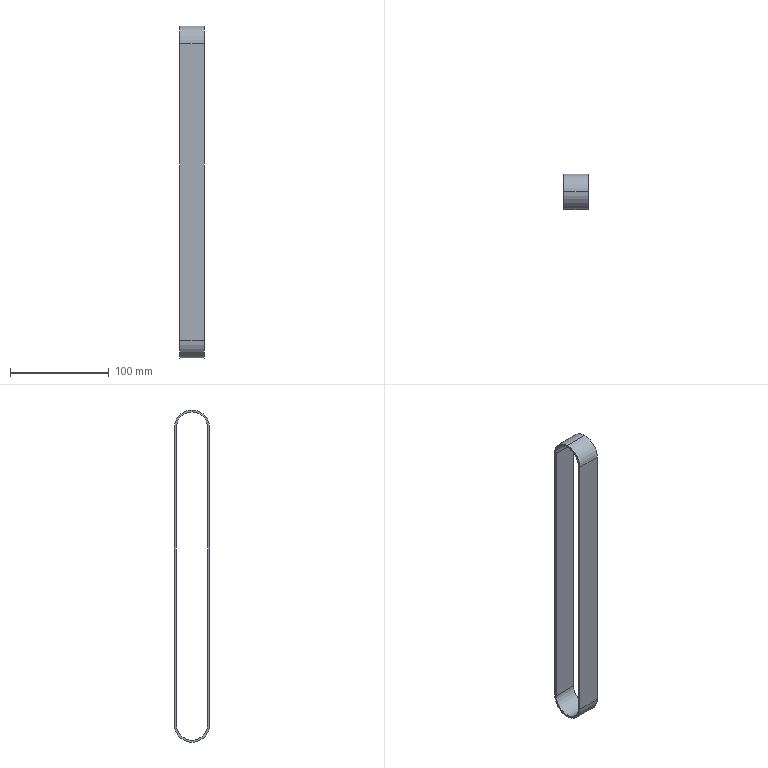Component | SolidWorks | RearConveyorLine,Width27mm-1 | 1 solid | 12 faces | box 25 x 35.84 x 335.84 mm | volume 35316 mm3 | cylinder 6 | plane 6 | commonest cylinder face diameters 31.84 x3 35.84 x3
build123d program:
from build123d import *

# Parameters (mm, degrees)
BOSS_EXTRUDE1_DEPTH = 12.5


with BuildPart() as part:
    # Sketch1 → Boss-Extrude1 (new, symmetric)
    with BuildSketch(Plane(origin=(0, 0, 0), x_dir=(0, 0, -1), z_dir=(1, 0, 0))):
        with BuildLine():
            Line((150, -17.92), (-150, -17.92))
            ThreePointArc((-150, -17.92), (-167.92, 0), (-150, 17.92))
            Line((-150, 17.92), (150, 17.92))
            ThreePointArc((150, 17.92), (167.92, 0), (150, -17.92))
        make_face()
        with BuildLine():
            Line((150, -15.92), (-150, -15.92))
            ThreePointArc((-150, -15.92), (-165.92, 0), (-150, 15.92))
            Line((-150, 15.92), (150, 15.92))
            ThreePointArc((150, 15.92), (165.92, 0), (150, -15.92))
        make_face(mode=Mode.SUBTRACT)
    extrude(amount=BOSS_EXTRUDE1_DEPTH, both=True)


solid = part.part

# Placed as in the assembly
solid = solid.moved(Location((21.5, 0, 0), (0, 0, 0)))
STEP:
#1=COLOUR_RGB('',0.7922,0.8196,0.9333);
#2=FILL_AREA_STYLE_COLOUR('',#1);
#3=FILL_AREA_STYLE('',(#2));
#4=SURFACE_STYLE_FILL_AREA(#3);
#5=SURFACE_SIDE_STYLE('',(#4));
#6=SURFACE_STYLE_USAGE(.BOTH.,#5);
#7=PRESENTATION_STYLE_ASSIGNMENT((#6));
#8=CARTESIAN_POINT('',(1.339,0.6268,5.906));
#9=VERTEX_POINT('',#8);
#10=CARTESIAN_POINT('',(1.339,-0.,6.532));
#11=VERTEX_POINT('',#10);
#12=CARTESIAN_POINT('',(1.339,-0.,5.906));
#13=DIRECTION('',(1.,0.,0.));
#14=DIRECTION('',(0.,0.,-1.));
#15=AXIS2_PLACEMENT_3D('',#12,#13,#14);
#16=CIRCLE('',#15,0.6268);
#17=EDGE_CURVE('',#9,#11,#16,.T.);
#18=ORIENTED_EDGE('',*,*,#17,.T.);
#19=CARTESIAN_POINT('',(0.3543,-0.,6.532));
#20=VERTEX_POINT('',#19);
#21=CARTESIAN_POINT('',(1.339,-0.,6.532));
#22=DIRECTION('',(-1.,0.,0.));
#23=VECTOR('',#22,39.37);
#24=LINE('',#21,#23);
#25=EDGE_CURVE('',#11,#20,#24,.T.);
#26=ORIENTED_EDGE('',*,*,#25,.T.);
#27=CARTESIAN_POINT('',(0.3543,0.6268,5.906));
#28=VERTEX_POINT('',#27);
#29=CARTESIAN_POINT('',(0.3543,-0.,5.906));
#30=DIRECTION('',(1.,0.,0.));
#31=DIRECTION('',(0.,0.,-1.));
#32=AXIS2_PLACEMENT_3D('',#29,#30,#31);
#33=CIRCLE('',#32,0.6268);
#34=EDGE_CURVE('',#28,#20,#33,.T.);
#35=ORIENTED_EDGE('',*,*,#34,.F.);
#36=CARTESIAN_POINT('',(1.339,0.6268,5.906));
#37=DIRECTION('',(-1.,0.,0.));
#38=VECTOR('',#37,39.37);
#39=LINE('',#36,#38);
#40=EDGE_CURVE('',#9,#28,#39,.T.);
#41=ORIENTED_EDGE('',*,*,#40,.F.);
#42=EDGE_LOOP('',(#18,#26,#35,#41));
#43=FACE_OUTER_BOUND('',#42,.T.);
#44=CARTESIAN_POINT('',(1.339,-0.,5.906));
#45=DIRECTION('',(-1.,0.,0.));
#46=DIRECTION('',(0.,0.,1.));
#47=AXIS2_PLACEMENT_3D('',#44,#45,#46);
#48=CYLINDRICAL_SURFACE('',#47,0.6268);
#49=ADVANCED_FACE('',(#43),#48,.F.);
#50=CARTESIAN_POINT('',(1.339,-0.,6.611));
#51=VERTEX_POINT('',#50);
#52=CARTESIAN_POINT('',(1.339,-0.7055,5.906));
#53=VERTEX_POINT('',#52);
#54=CARTESIAN_POINT('',(1.339,-0.,5.906));
#55=DIRECTION('',(1.,0.,0.));
#56=DIRECTION('',(0.,0.,-1.));
#57=AXIS2_PLACEMENT_3D('',#54,#55,#56);
#58=CIRCLE('',#57,0.7055);
#59=EDGE_CURVE('',#51,#53,#58,.T.);
#60=ORIENTED_EDGE('',*,*,#59,.F.);
#61=CARTESIAN_POINT('',(0.3543,-0.,6.611));
#62=VERTEX_POINT('',#61);
#63=CARTESIAN_POINT('',(1.339,-0.,6.611));
#64=DIRECTION('',(-1.,0.,0.));
#65=VECTOR('',#64,39.37);
#66=LINE('',#63,#65);
#67=EDGE_CURVE('',#51,#62,#66,.T.);
#68=ORIENTED_EDGE('',*,*,#67,.T.);
#69=CARTESIAN_POINT('',(0.3543,-0.7055,5.906));
#70=VERTEX_POINT('',#69);
#71=CARTESIAN_POINT('',(0.3543,-0.,5.906));
#72=DIRECTION('',(1.,0.,0.));
#73=DIRECTION('',(0.,0.,-1.));
#74=AXIS2_PLACEMENT_3D('',#71,#72,#73);
#75=CIRCLE('',#74,0.7055);
#76=EDGE_CURVE('',#62,#70,#75,.T.);
#77=ORIENTED_EDGE('',*,*,#76,.T.);
#78=CARTESIAN_POINT('',(1.339,-0.7055,5.906));
#79=DIRECTION('',(-1.,0.,0.));
#80=VECTOR('',#79,39.37);
#81=LINE('',#78,#80);
#82=EDGE_CURVE('',#53,#70,#81,.T.);
#83=ORIENTED_EDGE('',*,*,#82,.F.);
#84=EDGE_LOOP('',(#60,#68,#77,#83));
#85=FACE_OUTER_BOUND('',#84,.T.);
#86=CARTESIAN_POINT('',(1.339,-0.,5.906));
#87=DIRECTION('',(-1.,0.,0.));
#88=DIRECTION('',(0.,0.,1.));
#89=AXIS2_PLACEMENT_3D('',#86,#87,#88);
#90=CYLINDRICAL_SURFACE('',#89,0.7055);
#91=ADVANCED_FACE('',(#85),#90,.T.);
#92=CARTESIAN_POINT('',(1.339,-0.7055,-5.906));
#93=VERTEX_POINT('',#92);
#94=CARTESIAN_POINT('',(1.339,0.7055,-5.906));
#95=VERTEX_POINT('',#94);
#96=CARTESIAN_POINT('',(1.339,0.,-5.906));
#97=DIRECTION('',(1.,0.,0.));
#98=DIRECTION('',(0.,0.,-1.));
#99=AXIS2_PLACEMENT_3D('',#96,#97,#98);
#100=CIRCLE('',#99,0.7055);
#101=EDGE_CURVE('',#93,#95,#100,.T.);
#102=ORIENTED_EDGE('',*,*,#101,.T.);
#103=CARTESIAN_POINT('',(1.339,0.7055,5.906));
#104=VERTEX_POINT('',#103);
#105=CARTESIAN_POINT('',(1.339,0.7055,-5.906));
#106=DIRECTION('',(0.,-0.,1.));
#107=VECTOR('',#106,39.37);
#108=LINE('',#105,#107);
#109=EDGE_CURVE('',#95,#104,#108,.T.);
#110=ORIENTED_EDGE('',*,*,#109,.T.);
#111=CARTESIAN_POINT('',(1.339,-0.,5.906));
#112=DIRECTION('',(1.,0.,0.));
#113=DIRECTION('',(0.,0.,-1.));
#114=AXIS2_PLACEMENT_3D('',#111,#112,#113);
#115=CIRCLE('',#114,0.7055);
#116=EDGE_CURVE('',#104,#51,#115,.T.);
#117=ORIENTED_EDGE('',*,*,#116,.T.);
#118=ORIENTED_EDGE('',*,*,#59,.T.);
#119=CARTESIAN_POINT('',(1.339,-0.7055,-5.906));
#120=DIRECTION('',(0.,0.,-1.));
#121=VECTOR('',#120,39.37);
#122=LINE('',#119,#121);
#123=EDGE_CURVE('',#53,#93,#122,.T.);
#124=ORIENTED_EDGE('',*,*,#123,.T.);
#125=EDGE_LOOP('',(#102,#110,#117,#118,#124));
#126=FACE_OUTER_BOUND('',#125,.T.);
#127=CARTESIAN_POINT('',(1.339,0.6268,-5.906));
#128=VERTEX_POINT('',#127);
#129=CARTESIAN_POINT('',(1.339,0.6268,-5.906));
#130=DIRECTION('',(0.,-0.,1.));
#131=VECTOR('',#130,39.37);
#132=LINE('',#129,#131);
#133=EDGE_CURVE('',#128,#9,#132,.T.);
#134=ORIENTED_EDGE('',*,*,#133,.F.);
#135=CARTESIAN_POINT('',(1.339,-0.6268,-5.906));
#136=VERTEX_POINT('',#135);
#137=CARTESIAN_POINT('',(1.339,0.,-5.906));
#138=DIRECTION('',(1.,0.,0.));
#139=DIRECTION('',(0.,0.,-1.));
#140=AXIS2_PLACEMENT_3D('',#137,#138,#139);
#141=CIRCLE('',#140,0.6268);
#142=EDGE_CURVE('',#136,#128,#141,.T.);
#143=ORIENTED_EDGE('',*,*,#142,.F.);
#144=CARTESIAN_POINT('',(1.339,-0.6268,5.906));
#145=VERTEX_POINT('',#144);
#146=CARTESIAN_POINT('',(1.339,-0.6268,-5.906));
#147=DIRECTION('',(0.,0.,-1.));
#148=VECTOR('',#147,39.37);
#149=LINE('',#146,#148);
#150=EDGE_CURVE('',#145,#136,#149,.T.);
#151=ORIENTED_EDGE('',*,*,#150,.F.);
#152=CARTESIAN_POINT('',(1.339,-0.,5.906));
#153=DIRECTION('',(1.,0.,0.));
#154=DIRECTION('',(0.,0.,-1.));
#155=AXIS2_PLACEMENT_3D('',#152,#153,#154);
#156=CIRCLE('',#155,0.6268);
#157=EDGE_CURVE('',#11,#145,#156,.T.);
#158=ORIENTED_EDGE('',*,*,#157,.F.);
#159=ORIENTED_EDGE('',*,*,#17,.F.);
#160=EDGE_LOOP('',(#134,#143,#151,#158,#159));
#161=FACE_BOUND('',#160,.T.);
#162=CARTESIAN_POINT('',(1.339,0.,-5.906));
#163=DIRECTION('',(1.,0.,0.));
#164=DIRECTION('',(0.,0.,-1.));
#165=AXIS2_PLACEMENT_3D('',#162,#163,#164);
#166=PLANE('',#165);
#167=ADVANCED_FACE('',(#126,#161),#166,.T.);
#168=CARTESIAN_POINT('',(0.3543,-0.7055,-5.906));
#169=VERTEX_POINT('',#168);
#170=CARTESIAN_POINT('',(0.3543,0.7055,-5.906));
#171=VERTEX_POINT('',#170);
#172=CARTESIAN_POINT('',(0.3543,0.,-5.906));
#173=DIRECTION('',(1.,0.,0.));
#174=DIRECTION('',(0.,0.,-1.));
#175=AXIS2_PLACEMENT_3D('',#172,#173,#174);
#176=CIRCLE('',#175,0.7055);
#177=EDGE_CURVE('',#169,#171,#176,.T.);
#178=ORIENTED_EDGE('',*,*,#177,.F.);
#179=CARTESIAN_POINT('',(0.3543,-0.7055,-5.906));
#180=DIRECTION('',(0.,0.,-1.));
#181=VECTOR('',#180,39.37);
#182=LINE('',#179,#181);
#183=EDGE_CURVE('',#70,#169,#182,.T.);
#184=ORIENTED_EDGE('',*,*,#183,.F.);
#185=ORIENTED_EDGE('',*,*,#76,.F.);
#186=CARTESIAN_POINT('',(0.3543,0.7055,5.906));
#187=VERTEX_POINT('',#186);
#188=CARTESIAN_POINT('',(0.3543,-0.,5.906));
#189=DIRECTION('',(1.,0.,0.));
#190=DIRECTION('',(0.,0.,-1.));
#191=AXIS2_PLACEMENT_3D('',#188,#189,#190);
#192=CIRCLE('',#191,0.7055);
#193=EDGE_CURVE('',#187,#62,#192,.T.);
#194=ORIENTED_EDGE('',*,*,#193,.F.);
#195=CARTESIAN_POINT('',(0.3543,0.7055,-5.906));
#196=DIRECTION('',(0.,-0.,1.));
#197=VECTOR('',#196,39.37);
#198=LINE('',#195,#197);
#199=EDGE_CURVE('',#171,#187,#198,.T.);
#200=ORIENTED_EDGE('',*,*,#199,.F.);
#201=EDGE_LOOP('',(#178,#184,#185,#194,#200));
#202=FACE_OUTER_BOUND('',#201,.T.);
#203=CARTESIAN_POINT('',(0.3543,-0.6268,-5.906));
#204=VERTEX_POINT('',#203);
#205=CARTESIAN_POINT('',(0.3543,0.6268,-5.906));
#206=VERTEX_POINT('',#205);
#207=CARTESIAN_POINT('',(0.3543,0.,-5.906));
#208=DIRECTION('',(1.,0.,0.));
#209=DIRECTION('',(0.,0.,-1.));
#210=AXIS2_PLACEMENT_3D('',#207,#208,#209);
#211=CIRCLE('',#210,0.6268);
#212=EDGE_CURVE('',#204,#206,#211,.T.);
#213=ORIENTED_EDGE('',*,*,#212,.T.);
#214=CARTESIAN_POINT('',(0.3543,0.6268,-5.906));
#215=DIRECTION('',(0.,-0.,1.));
#216=VECTOR('',#215,39.37);
#217=LINE('',#214,#216);
#218=EDGE_CURVE('',#206,#28,#217,.T.);
#219=ORIENTED_EDGE('',*,*,#218,.T.);
#220=ORIENTED_EDGE('',*,*,#34,.T.);
#221=CARTESIAN_POINT('',(0.3543,-0.6268,5.906));
#222=VERTEX_POINT('',#221);
#223=CARTESIAN_POINT('',(0.3543,-0.,5.906));
#224=DIRECTION('',(1.,0.,0.));
#225=DIRECTION('',(0.,0.,-1.));
#226=AXIS2_PLACEMENT_3D('',#223,#224,#225);
#227=CIRCLE('',#226,0.6268);
#228=EDGE_CURVE('',#20,#222,#227,.T.);
#229=ORIENTED_EDGE('',*,*,#228,.T.);
#230=CARTESIAN_POINT('',(0.3543,-0.6268,-5.906));
#231=DIRECTION('',(0.,0.,-1.));
#232=VECTOR('',#231,39.37);
#233=LINE('',#230,#232);
#234=EDGE_CURVE('',#222,#204,#233,.T.);
#235=ORIENTED_EDGE('',*,*,#234,.T.);
#236=EDGE_LOOP('',(#213,#219,#220,#229,#235));
#237=FACE_BOUND('',#236,.T.);
#238=CARTESIAN_POINT('',(0.3543,0.,-5.906));
#239=DIRECTION('',(1.,0.,0.));
#240=DIRECTION('',(0.,0.,-1.));
#241=AXIS2_PLACEMENT_3D('',#238,#239,#240);
#242=PLANE('',#241);
#243=ADVANCED_FACE('',(#202,#237),#242,.F.);
#244=ORIENTED_EDGE('',*,*,#177,.T.);
#245=CARTESIAN_POINT('',(1.339,0.7055,-5.906));
#246=DIRECTION('',(-1.,0.,0.));
#247=VECTOR('',#246,39.37);
#248=LINE('',#245,#247);
#249=EDGE_CURVE('',#95,#171,#248,.T.);
#250=ORIENTED_EDGE('',*,*,#249,.F.);
#251=ORIENTED_EDGE('',*,*,#101,.F.);
#252=CARTESIAN_POINT('',(1.339,-0.7055,-5.906));
#253=DIRECTION('',(-1.,0.,0.));
#254=VECTOR('',#253,39.37);
#255=LINE('',#252,#254);
#256=EDGE_CURVE('',#93,#169,#255,.T.);
#257=ORIENTED_EDGE('',*,*,#256,.T.);
#258=EDGE_LOOP('',(#244,#250,#251,#257));
#259=FACE_OUTER_BOUND('',#258,.T.);
#260=CARTESIAN_POINT('',(1.339,0.,-5.906));
#261=DIRECTION('',(-1.,0.,0.));
#262=DIRECTION('',(0.,0.,1.));
#263=AXIS2_PLACEMENT_3D('',#260,#261,#262);
#264=CYLINDRICAL_SURFACE('',#263,0.7055);
#265=ADVANCED_FACE('',(#259),#264,.T.);
#266=ORIENTED_EDGE('',*,*,#199,.T.);
#267=CARTESIAN_POINT('',(1.339,0.7055,5.906));
#268=DIRECTION('',(-1.,0.,0.));
#269=VECTOR('',#268,39.37);
#270=LINE('',#267,#269);
#271=EDGE_CURVE('',#104,#187,#270,.T.);
#272=ORIENTED_EDGE('',*,*,#271,.F.);
#273=ORIENTED_EDGE('',*,*,#109,.F.);
#274=ORIENTED_EDGE('',*,*,#249,.T.);
#275=EDGE_LOOP('',(#266,#272,#273,#274));
#276=FACE_OUTER_BOUND('',#275,.T.);
#277=CARTESIAN_POINT('',(1.339,0.7055,-5.906));
#278=DIRECTION('',(0.,-1.,-0.));
#279=DIRECTION('',(0.,0.,-1.));
#280=AXIS2_PLACEMENT_3D('',#277,#278,#279);
#281=PLANE('',#280);
#282=ADVANCED_FACE('',(#276),#281,.F.);
#283=ORIENTED_EDGE('',*,*,#67,.F.);
#284=ORIENTED_EDGE('',*,*,#116,.F.);
#285=ORIENTED_EDGE('',*,*,#271,.T.);
#286=ORIENTED_EDGE('',*,*,#193,.T.);
#287=EDGE_LOOP('',(#283,#284,#285,#286));
#288=FACE_OUTER_BOUND('',#287,.T.);
#289=CARTESIAN_POINT('',(1.339,-0.,5.906));
#290=DIRECTION('',(-1.,0.,0.));
#291=DIRECTION('',(0.,0.,1.));
#292=AXIS2_PLACEMENT_3D('',#289,#290,#291);
#293=CYLINDRICAL_SURFACE('',#292,0.7055);
#294=ADVANCED_FACE('',(#288),#293,.T.);
#295=ORIENTED_EDGE('',*,*,#183,.T.);
#296=ORIENTED_EDGE('',*,*,#256,.F.);
#297=ORIENTED_EDGE('',*,*,#123,.F.);
#298=ORIENTED_EDGE('',*,*,#82,.T.);
#299=EDGE_LOOP('',(#295,#296,#297,#298));
#300=FACE_OUTER_BOUND('',#299,.T.);
#301=CARTESIAN_POINT('',(1.339,-0.7055,-5.906));
#302=DIRECTION('',(0.,1.,0.));
#303=DIRECTION('',(0.,-0.,1.));
#304=AXIS2_PLACEMENT_3D('',#301,#302,#303);
#305=PLANE('',#304);
#306=ADVANCED_FACE('',(#300),#305,.F.);
#307=ORIENTED_EDGE('',*,*,#212,.F.);
#308=CARTESIAN_POINT('',(1.339,-0.6268,-5.906));
#309=DIRECTION('',(-1.,0.,0.));
#310=VECTOR('',#309,39.37);
#311=LINE('',#308,#310);
#312=EDGE_CURVE('',#136,#204,#311,.T.);
#313=ORIENTED_EDGE('',*,*,#312,.F.);
#314=ORIENTED_EDGE('',*,*,#142,.T.);
#315=CARTESIAN_POINT('',(1.339,0.6268,-5.906));
#316=DIRECTION('',(-1.,0.,0.));
#317=VECTOR('',#316,39.37);
#318=LINE('',#315,#317);
#319=EDGE_CURVE('',#128,#206,#318,.T.);
#320=ORIENTED_EDGE('',*,*,#319,.T.);
#321=EDGE_LOOP('',(#307,#313,#314,#320));
#322=FACE_OUTER_BOUND('',#321,.T.);
#323=CARTESIAN_POINT('',(1.339,0.,-5.906));
#324=DIRECTION('',(-1.,0.,0.));
#325=DIRECTION('',(0.,0.,1.));
#326=AXIS2_PLACEMENT_3D('',#323,#324,#325);
#327=CYLINDRICAL_SURFACE('',#326,0.6268);
#328=ADVANCED_FACE('',(#322),#327,.F.);
#329=ORIENTED_EDGE('',*,*,#218,.F.);
#330=ORIENTED_EDGE('',*,*,#319,.F.);
#331=ORIENTED_EDGE('',*,*,#133,.T.);
#332=ORIENTED_EDGE('',*,*,#40,.T.);
#333=EDGE_LOOP('',(#329,#330,#331,#332));
#334=FACE_OUTER_BOUND('',#333,.T.);
#335=CARTESIAN_POINT('',(1.339,0.6268,-5.906));
#336=DIRECTION('',(0.,-1.,-0.));
#337=DIRECTION('',(0.,0.,-1.));
#338=AXIS2_PLACEMENT_3D('',#335,#336,#337);
#339=PLANE('',#338);
#340=ADVANCED_FACE('',(#334),#339,.T.);
#341=ORIENTED_EDGE('',*,*,#25,.F.);
#342=ORIENTED_EDGE('',*,*,#157,.T.);
#343=CARTESIAN_POINT('',(1.339,-0.6268,5.906));
#344=DIRECTION('',(-1.,0.,0.));
#345=VECTOR('',#344,39.37);
#346=LINE('',#343,#345);
#347=EDGE_CURVE('',#145,#222,#346,.T.);
#348=ORIENTED_EDGE('',*,*,#347,.T.);
#349=ORIENTED_EDGE('',*,*,#228,.F.);
#350=EDGE_LOOP('',(#341,#342,#348,#349));
#351=FACE_OUTER_BOUND('',#350,.T.);
#352=CARTESIAN_POINT('',(1.339,-0.,5.906));
#353=DIRECTION('',(-1.,0.,0.));
#354=DIRECTION('',(0.,0.,1.));
#355=AXIS2_PLACEMENT_3D('',#352,#353,#354);
#356=CYLINDRICAL_SURFACE('',#355,0.6268);
#357=ADVANCED_FACE('',(#351),#356,.F.);
#358=ORIENTED_EDGE('',*,*,#234,.F.);
#359=ORIENTED_EDGE('',*,*,#347,.F.);
#360=ORIENTED_EDGE('',*,*,#150,.T.);
#361=ORIENTED_EDGE('',*,*,#312,.T.);
#362=EDGE_LOOP('',(#358,#359,#360,#361));
#363=FACE_OUTER_BOUND('',#362,.T.);
#364=CARTESIAN_POINT('',(1.339,-0.6268,-5.906));
#365=DIRECTION('',(0.,1.,0.));
#366=DIRECTION('',(0.,-0.,1.));
#367=AXIS2_PLACEMENT_3D('',#364,#365,#366);
#368=PLANE('',#367);
#369=ADVANCED_FACE('',(#363),#368,.T.);
#370=CLOSED_SHELL('',(#49,#91,#167,#243,#265,#282,#294,#306,#328,#340,#357,#369));
#371=MANIFOLD_SOLID_BREP('',#370);
#372=STYLED_ITEM('',(#7),#371);
#373=PRESENTATION_LAYER_ASSIGNMENT('','',(#372));
#374=(LENGTH_UNIT()NAMED_UNIT(*)SI_UNIT($,.METRE.));
#375=LENGTH_MEASURE_WITH_UNIT(LENGTH_MEASURE(0.0254),#374);
#376=DIMENSIONAL_EXPONENTS(1.,0.,0.,0.,0.,0.,0.);
#377=(CONVERSION_BASED_UNIT('',#375)LENGTH_UNIT()NAMED_UNIT(#376));
#378=UNCERTAINTY_MEASURE_WITH_UNIT(LENGTH_MEASURE(0.00001),#377,'','');
#379=(NAMED_UNIT(*)PLANE_ANGLE_UNIT()SI_UNIT($,.RADIAN.));
#380=(NAMED_UNIT(*)SI_UNIT($,.STERADIAN.)SOLID_ANGLE_UNIT());
#381=(GEOMETRIC_REPRESENTATION_CONTEXT(3)GLOBAL_UNCERTAINTY_ASSIGNED_CONTEXT((#378))GLOBAL_UNIT_ASSIGNED_CONTEXT((#377,#379,#380))REPRESENTATION_CONTEXT('',''));
#382=MECHANICAL_DESIGN_GEOMETRIC_PRESENTATION_REPRESENTATION('',(#372),#381);
#383=CARTESIAN_POINT('',(0.,0.,0.));
#384=DIRECTION('',(0.,0.,1.));
#385=DIRECTION('',(1.,0.,0.));
#386=AXIS2_PLACEMENT_3D('',#383,#384,#385);
#387=(LENGTH_UNIT()NAMED_UNIT(*)SI_UNIT($,.METRE.));
#388=LENGTH_MEASURE_WITH_UNIT(LENGTH_MEASURE(0.0254),#387);
#389=DIMENSIONAL_EXPONENTS(1.,0.,0.,0.,0.,0.,0.);
#390=(CONVERSION_BASED_UNIT('',#388)LENGTH_UNIT()NAMED_UNIT(#389));
#391=UNCERTAINTY_MEASURE_WITH_UNIT(LENGTH_MEASURE(0.00001),#390,'','');
#392=(NAMED_UNIT(*)PLANE_ANGLE_UNIT()SI_UNIT($,.RADIAN.));
#393=(NAMED_UNIT(*)SI_UNIT($,.STERADIAN.)SOLID_ANGLE_UNIT());
#394=(GEOMETRIC_REPRESENTATION_CONTEXT(3)GLOBAL_UNCERTAINTY_ASSIGNED_CONTEXT((#391))GLOBAL_UNIT_ASSIGNED_CONTEXT((#390,#392,#393))REPRESENTATION_CONTEXT('',''));
#395=ADVANCED_BREP_SHAPE_REPRESENTATION('',(#371,#386),#394);